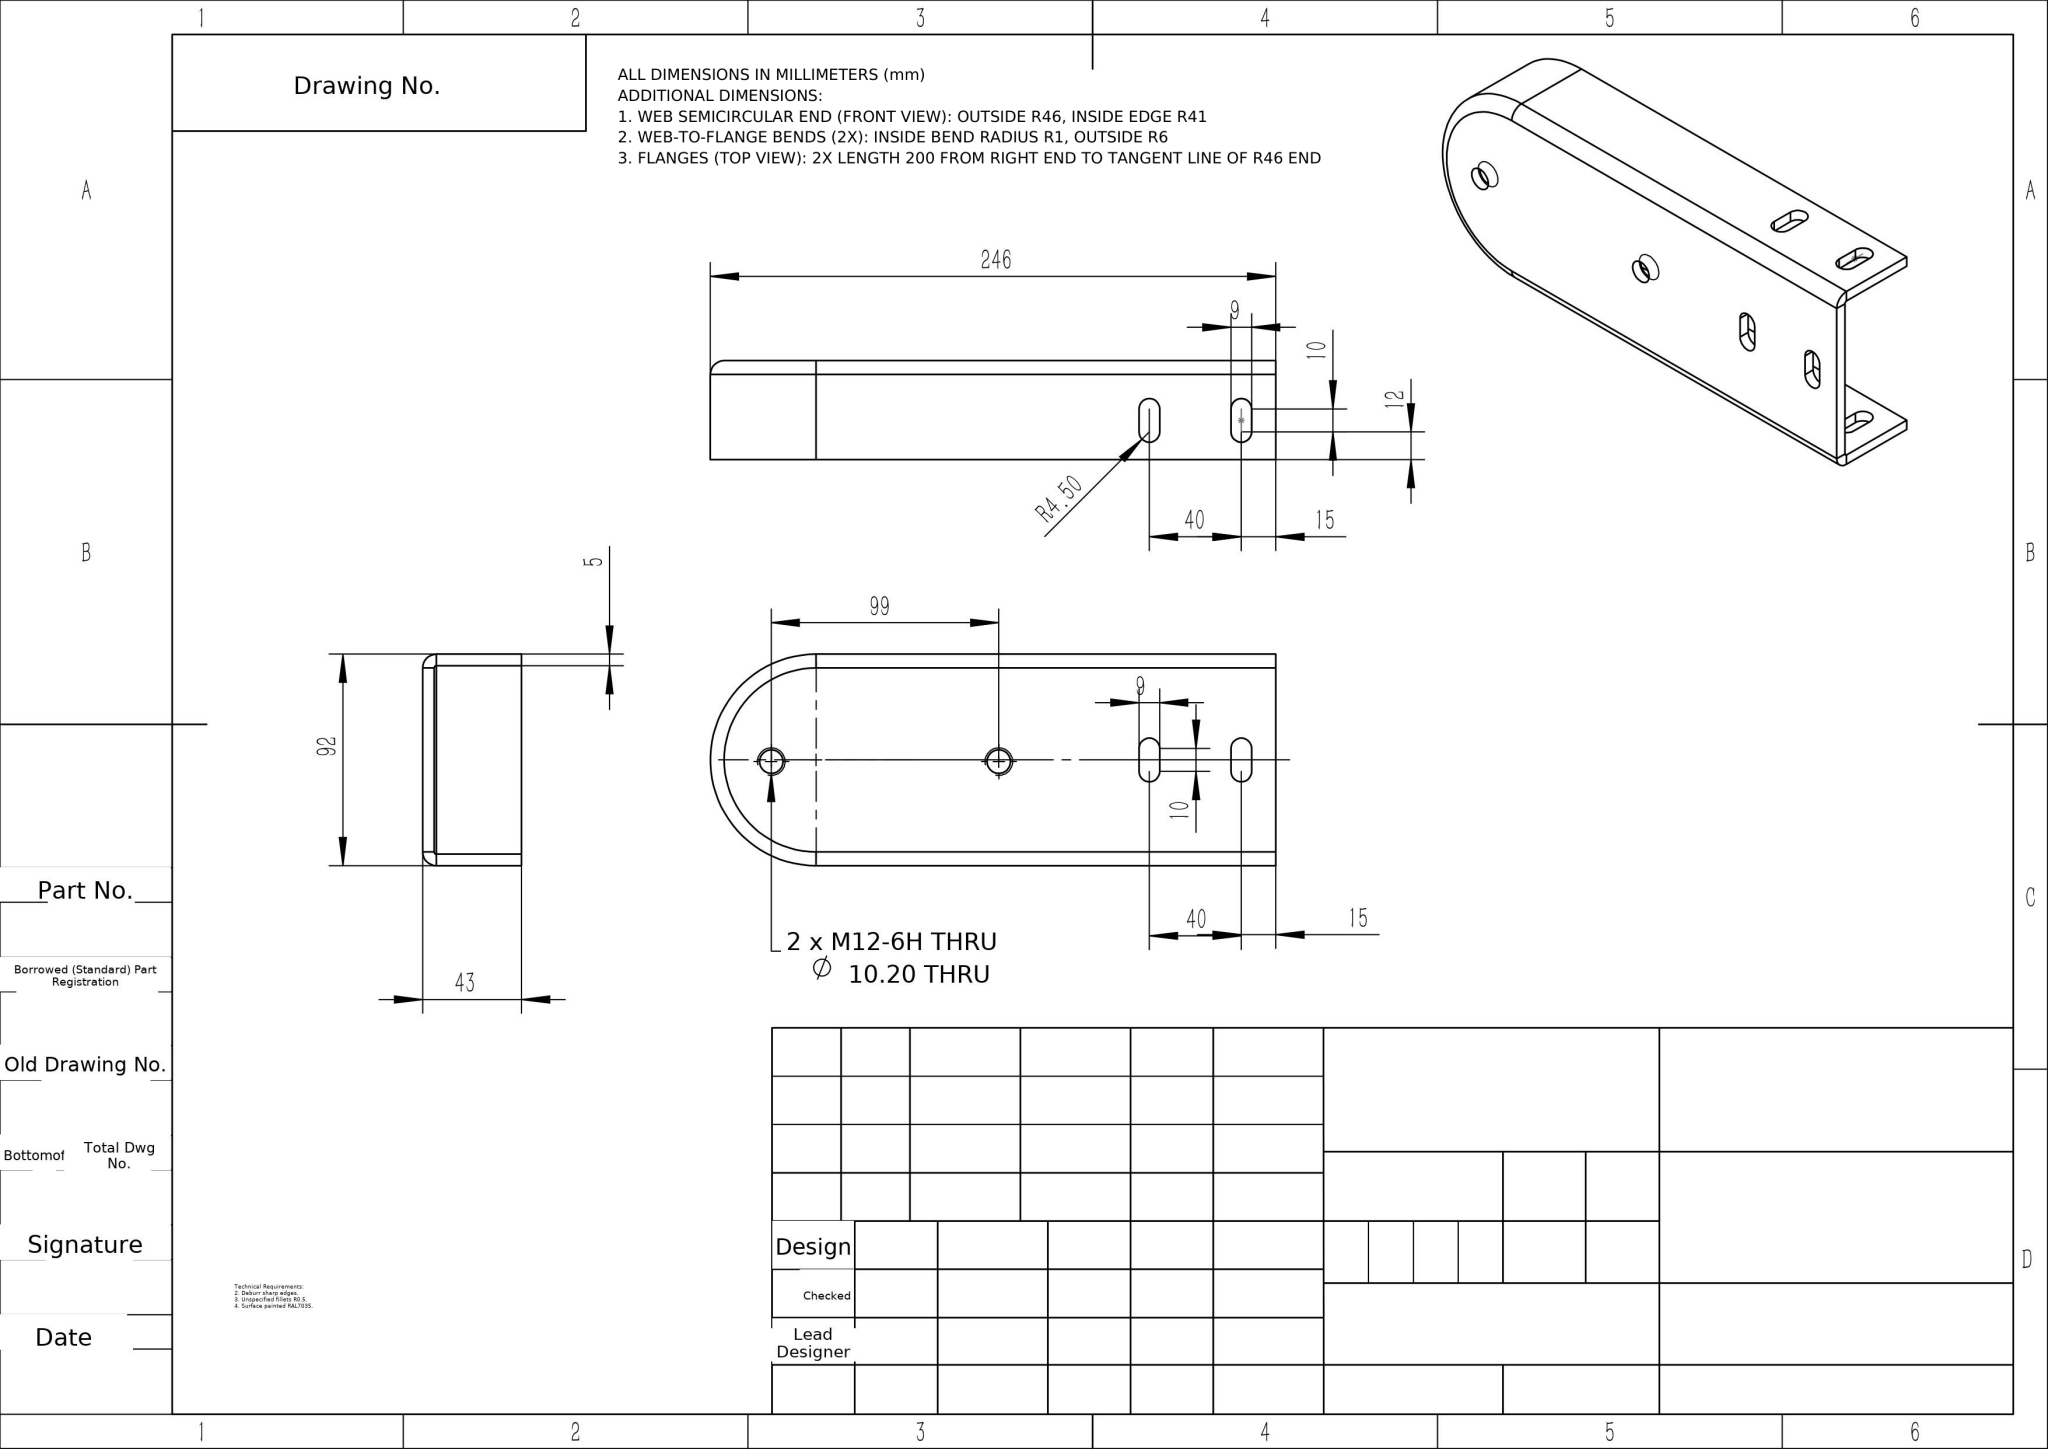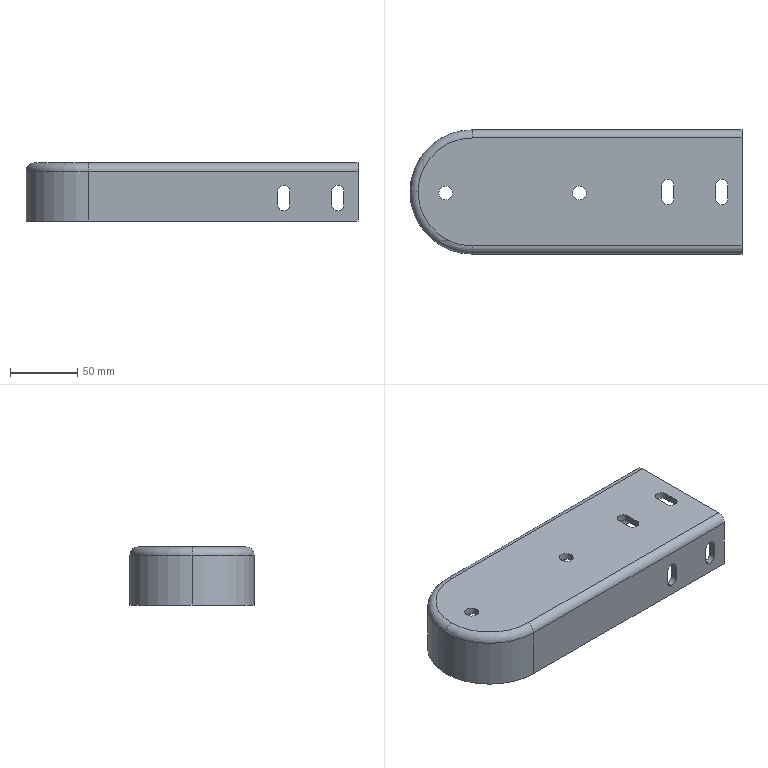Part | NX | mm | 1 solid | 58 faces | box 246 x 92 x 43 mm | volume 201098 mm3 | cylinder 28 | plane 26 | torus 4 | commonest cylinder face diameters 9 x16 10.2 x4 92 x2 82 x2 2 x2 12 x2